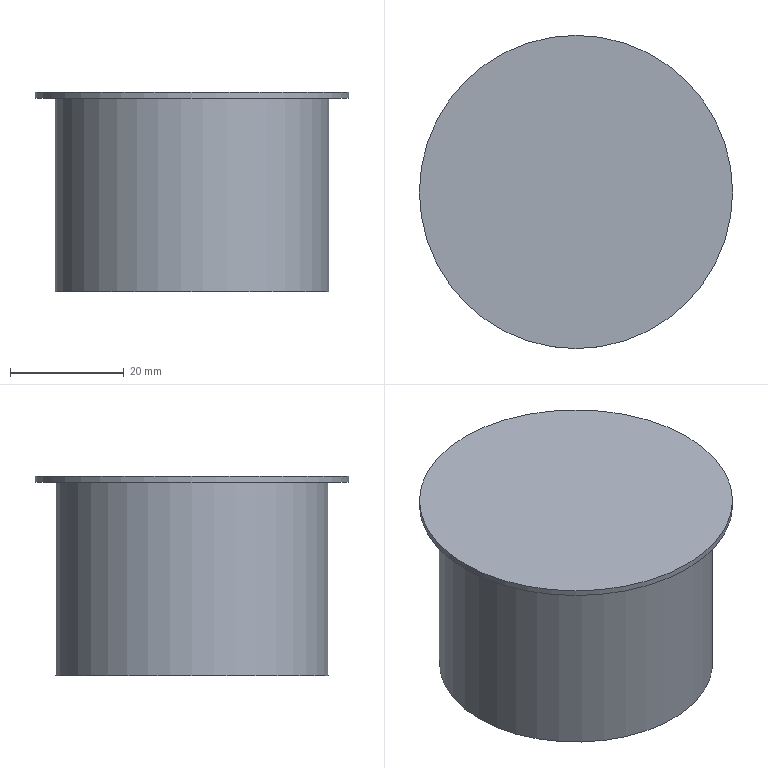Component | NX | MOUNT | 1 solid | 5 faces | box 55 x 55 x 35 mm | volume 63901 mm3 | plane 3 | cylinder 2 | commonest cylinder face diameters 48 x1 55 x1
STEP:
#1=CARTESIAN_POINT('',(0.,0.,0.));
#2=DIRECTION('',(0.,0.,1.));
#3=DIRECTION('',(1.,0.,0.));
#4=AXIS2_PLACEMENT_3D('',#1,#2,#3);
#5=CARTESIAN_POINT('',(-169.726,-83.,-35.));
#6=VERTEX_POINT('',#5);
#7=CARTESIAN_POINT('',(-145.726,-83.,-35.));
#8=DIRECTION('',(0.,0.,-1.));
#9=DIRECTION('',(-1.,0.,0.));
#10=AXIS2_PLACEMENT_3D('',#7,#8,#9);
#11=CIRCLE('',#10,24.);
#12=CARTESIAN_POINT('',(-145.726,-83.,-35.));
#13=DIRECTION('',(0.,0.,1.));
#14=DIRECTION('',(1.,0.,0.));
#15=AXIS2_PLACEMENT_3D('',#12,#13,#14);
#16=CYLINDRICAL_SURFACE('',#15,24.);
#17=CARTESIAN_POINT('',(9.425,0.));
#18=DIRECTION('',(-1.,0.));
#19=VECTOR('',#18,1.);
#20=LINE('',#17,#19);
#21=(GEOMETRIC_REPRESENTATION_CONTEXT(2)PARAMETRIC_REPRESENTATION_CONTEXT()REPRESENTATION_CONTEXT('',''));
#22=DEFINITIONAL_REPRESENTATION('',(#20),#21);
#23=PCURVE('',#16,#22);
#24=CARTESIAN_POINT('',(-145.726,-83.,-35.));
#25=DIRECTION('',(0.,0.,-1.));
#26=DIRECTION('',(-1.,0.,0.));
#27=AXIS2_PLACEMENT_3D('',#24,#25,#26);
#28=PLANE('',#27);
#29=CARTESIAN_POINT('',(0.,0.));
#30=DIRECTION('',(1.,0.));
#31=AXIS2_PLACEMENT_2D('',#29,#30);
#32=CIRCLE('',#31,24.);
#33=(GEOMETRIC_REPRESENTATION_CONTEXT(2)PARAMETRIC_REPRESENTATION_CONTEXT()REPRESENTATION_CONTEXT('',''));
#34=DEFINITIONAL_REPRESENTATION('',(#32),#33);
#35=PCURVE('',#28,#34);
#36=SURFACE_CURVE('',#11,(#23,#35),.PCURVE_S1.);
#37=EDGE_CURVE('',#6,#6,#36,.T.);
#38=ORIENTED_EDGE('',*,*,#37,.F.);
#39=CARTESIAN_POINT('',(-169.726,-83.,-1.));
#40=VERTEX_POINT('',#39);
#41=CARTESIAN_POINT('',(-169.726,-83.,-35.));
#42=CARTESIAN_POINT('',(-169.726,-83.,-1.));
#43=B_SPLINE_CURVE_WITH_KNOTS('',1,(#41,#42),.UNSPECIFIED.,.F.,.F.,(2,2),(0.,34.),.PIECEWISE_BEZIER_KNOTS.);
#44=CARTESIAN_POINT('',(9.425,0.));
#45=DIRECTION('',(0.,1.));
#46=VECTOR('',#45,1.);
#47=LINE('',#44,#46);
#48=(GEOMETRIC_REPRESENTATION_CONTEXT(2)PARAMETRIC_REPRESENTATION_CONTEXT()REPRESENTATION_CONTEXT('',''));
#49=DEFINITIONAL_REPRESENTATION('',(#47),#48);
#50=PCURVE('',#16,#49);
#51=CARTESIAN_POINT('',(3.142,0.));
#52=DIRECTION('',(0.,1.));
#53=VECTOR('',#52,1.);
#54=LINE('',#51,#53);
#55=(GEOMETRIC_REPRESENTATION_CONTEXT(2)PARAMETRIC_REPRESENTATION_CONTEXT()REPRESENTATION_CONTEXT('',''));
#56=DEFINITIONAL_REPRESENTATION('',(#54),#55);
#57=PCURVE('',#16,#56);
#58=SEAM_CURVE('',#43,(#50,#57),.PCURVE_S1.);
#59=EDGE_CURVE('',#6,#40,#58,.T.);
#60=ORIENTED_EDGE('',*,*,#59,.T.);
#61=CARTESIAN_POINT('',(-145.726,-83.,-1.));
#62=DIRECTION('',(0.,0.,-1.));
#63=DIRECTION('',(-1.,0.,0.));
#64=AXIS2_PLACEMENT_3D('',#61,#62,#63);
#65=CIRCLE('',#64,24.);
#66=CARTESIAN_POINT('',(9.425,34.));
#67=DIRECTION('',(-1.,0.));
#68=VECTOR('',#67,1.);
#69=LINE('',#66,#68);
#70=(GEOMETRIC_REPRESENTATION_CONTEXT(2)PARAMETRIC_REPRESENTATION_CONTEXT()REPRESENTATION_CONTEXT('',''));
#71=DEFINITIONAL_REPRESENTATION('',(#69),#70);
#72=PCURVE('',#16,#71);
#73=CARTESIAN_POINT('',(-145.726,-83.,-1.));
#74=DIRECTION('',(0.,0.,-1.));
#75=DIRECTION('',(-1.,0.,0.));
#76=AXIS2_PLACEMENT_3D('',#73,#74,#75);
#77=PLANE('',#76);
#78=CARTESIAN_POINT('',(0.,0.));
#79=DIRECTION('',(1.,0.));
#80=AXIS2_PLACEMENT_2D('',#78,#79);
#81=CIRCLE('',#80,24.);
#82=(GEOMETRIC_REPRESENTATION_CONTEXT(2)PARAMETRIC_REPRESENTATION_CONTEXT()REPRESENTATION_CONTEXT('',''));
#83=DEFINITIONAL_REPRESENTATION('',(#81),#82);
#84=PCURVE('',#77,#83);
#85=SURFACE_CURVE('',#65,(#72,#84),.PCURVE_S1.);
#86=EDGE_CURVE('',#40,#40,#85,.T.);
#87=ORIENTED_EDGE('',*,*,#86,.T.);
#88=ORIENTED_EDGE('',*,*,#59,.F.);
#89=EDGE_LOOP('',(#38,#60,#87,#88));
#90=FACE_BOUND('',#89,.T.);
#91=ADVANCED_FACE('',(#90),#16,.T.);
#92=ORIENTED_EDGE('',*,*,#37,.T.);
#93=EDGE_LOOP('',(#92));
#94=FACE_BOUND('',#93,.T.);
#95=ADVANCED_FACE('',(#94),#28,.T.);
#96=CARTESIAN_POINT('',(-173.226,-83.,-1.));
#97=VERTEX_POINT('',#96);
#98=CARTESIAN_POINT('',(-145.726,-83.,-1.));
#99=DIRECTION('',(0.,0.,-1.));
#100=DIRECTION('',(-1.,0.,0.));
#101=AXIS2_PLACEMENT_3D('',#98,#99,#100);
#102=CIRCLE('',#101,27.5);
#103=CARTESIAN_POINT('',(-145.726,-83.,-1.));
#104=DIRECTION('',(0.,0.,1.));
#105=DIRECTION('',(1.,0.,0.));
#106=AXIS2_PLACEMENT_3D('',#103,#104,#105);
#107=CYLINDRICAL_SURFACE('',#106,27.5);
#108=CARTESIAN_POINT('',(9.425,0.));
#109=DIRECTION('',(-1.,0.));
#110=VECTOR('',#109,1.);
#111=LINE('',#108,#110);
#112=(GEOMETRIC_REPRESENTATION_CONTEXT(2)PARAMETRIC_REPRESENTATION_CONTEXT()REPRESENTATION_CONTEXT('',''));
#113=DEFINITIONAL_REPRESENTATION('',(#111),#112);
#114=PCURVE('',#107,#113);
#115=CARTESIAN_POINT('',(0.,0.));
#116=DIRECTION('',(1.,0.));
#117=AXIS2_PLACEMENT_2D('',#115,#116);
#118=CIRCLE('',#117,27.5);
#119=(GEOMETRIC_REPRESENTATION_CONTEXT(2)PARAMETRIC_REPRESENTATION_CONTEXT()REPRESENTATION_CONTEXT('',''));
#120=DEFINITIONAL_REPRESENTATION('',(#118),#119);
#121=PCURVE('',#77,#120);
#122=SURFACE_CURVE('',#102,(#114,#121),.PCURVE_S1.);
#123=EDGE_CURVE('',#97,#97,#122,.T.);
#124=ORIENTED_EDGE('',*,*,#123,.F.);
#125=CARTESIAN_POINT('',(-173.226,-83.,0.));
#126=VERTEX_POINT('',#125);
#127=CARTESIAN_POINT('',(-173.226,-83.,-1.));
#128=CARTESIAN_POINT('',(-173.226,-83.,0.));
#129=B_SPLINE_CURVE_WITH_KNOTS('',1,(#127,#128),.UNSPECIFIED.,.F.,.F.,(2,2),(0.,1.),.PIECEWISE_BEZIER_KNOTS.);
#130=CARTESIAN_POINT('',(9.425,0.));
#131=DIRECTION('',(0.,1.));
#132=VECTOR('',#131,1.);
#133=LINE('',#130,#132);
#134=(GEOMETRIC_REPRESENTATION_CONTEXT(2)PARAMETRIC_REPRESENTATION_CONTEXT()REPRESENTATION_CONTEXT('',''));
#135=DEFINITIONAL_REPRESENTATION('',(#133),#134);
#136=PCURVE('',#107,#135);
#137=CARTESIAN_POINT('',(3.142,0.));
#138=DIRECTION('',(0.,1.));
#139=VECTOR('',#138,1.);
#140=LINE('',#137,#139);
#141=(GEOMETRIC_REPRESENTATION_CONTEXT(2)PARAMETRIC_REPRESENTATION_CONTEXT()REPRESENTATION_CONTEXT('',''));
#142=DEFINITIONAL_REPRESENTATION('',(#140),#141);
#143=PCURVE('',#107,#142);
#144=SEAM_CURVE('',#129,(#136,#143),.PCURVE_S1.);
#145=EDGE_CURVE('',#97,#126,#144,.T.);
#146=ORIENTED_EDGE('',*,*,#145,.T.);
#147=CARTESIAN_POINT('',(-145.726,-83.,0.));
#148=DIRECTION('',(0.,0.,-1.));
#149=DIRECTION('',(-1.,0.,0.));
#150=AXIS2_PLACEMENT_3D('',#147,#148,#149);
#151=CIRCLE('',#150,27.5);
#152=CARTESIAN_POINT('',(9.425,1.));
#153=DIRECTION('',(-1.,0.));
#154=VECTOR('',#153,1.);
#155=LINE('',#152,#154);
#156=(GEOMETRIC_REPRESENTATION_CONTEXT(2)PARAMETRIC_REPRESENTATION_CONTEXT()REPRESENTATION_CONTEXT('',''));
#157=DEFINITIONAL_REPRESENTATION('',(#155),#156);
#158=PCURVE('',#107,#157);
#159=CARTESIAN_POINT('',(-145.726,-83.,0.));
#160=DIRECTION('',(0.,0.,-1.));
#161=DIRECTION('',(-1.,0.,0.));
#162=AXIS2_PLACEMENT_3D('',#159,#160,#161);
#163=PLANE('',#162);
#164=CARTESIAN_POINT('',(0.,0.));
#165=DIRECTION('',(1.,0.));
#166=AXIS2_PLACEMENT_2D('',#164,#165);
#167=CIRCLE('',#166,27.5);
#168=(GEOMETRIC_REPRESENTATION_CONTEXT(2)PARAMETRIC_REPRESENTATION_CONTEXT()REPRESENTATION_CONTEXT('',''));
#169=DEFINITIONAL_REPRESENTATION('',(#167),#168);
#170=PCURVE('',#163,#169);
#171=SURFACE_CURVE('',#151,(#158,#170),.PCURVE_S1.);
#172=EDGE_CURVE('',#126,#126,#171,.T.);
#173=ORIENTED_EDGE('',*,*,#172,.T.);
#174=ORIENTED_EDGE('',*,*,#145,.F.);
#175=EDGE_LOOP('',(#124,#146,#173,#174));
#176=FACE_BOUND('',#175,.T.);
#177=ADVANCED_FACE('',(#176),#107,.T.);
#178=ORIENTED_EDGE('',*,*,#86,.F.);
#179=EDGE_LOOP('',(#178));
#180=FACE_BOUND('',#179,.T.);
#181=ORIENTED_EDGE('',*,*,#123,.T.);
#182=EDGE_LOOP('',(#181));
#183=FACE_BOUND('',#182,.T.);
#184=ADVANCED_FACE('',(#180,#183),#77,.T.);
#185=ORIENTED_EDGE('',*,*,#172,.F.);
#186=EDGE_LOOP('',(#185));
#187=FACE_BOUND('',#186,.T.);
#188=ADVANCED_FACE('',(#187),#163,.F.);
#189=CLOSED_SHELL('',(#91,#95,#177,#184,#188));
#190=MANIFOLD_SOLID_BREP('',#189);
#191=(LENGTH_UNIT()NAMED_UNIT(*)SI_UNIT(.MILLI.,.METRE.));
#192=UNCERTAINTY_MEASURE_WITH_UNIT(LENGTH_MEASURE(0.00001),#191,'','');
#193=(NAMED_UNIT(*)PLANE_ANGLE_UNIT()SI_UNIT($,.RADIAN.));
#194=(NAMED_UNIT(*)SI_UNIT($,.STERADIAN.)SOLID_ANGLE_UNIT());
#195=(GEOMETRIC_REPRESENTATION_CONTEXT(3)GLOBAL_UNCERTAINTY_ASSIGNED_CONTEXT((#192))GLOBAL_UNIT_ASSIGNED_CONTEXT((#191,#193,#194))REPRESENTATION_CONTEXT('',''));
#196=ADVANCED_BREP_SHAPE_REPRESENTATION('',(#4,#190),#195);